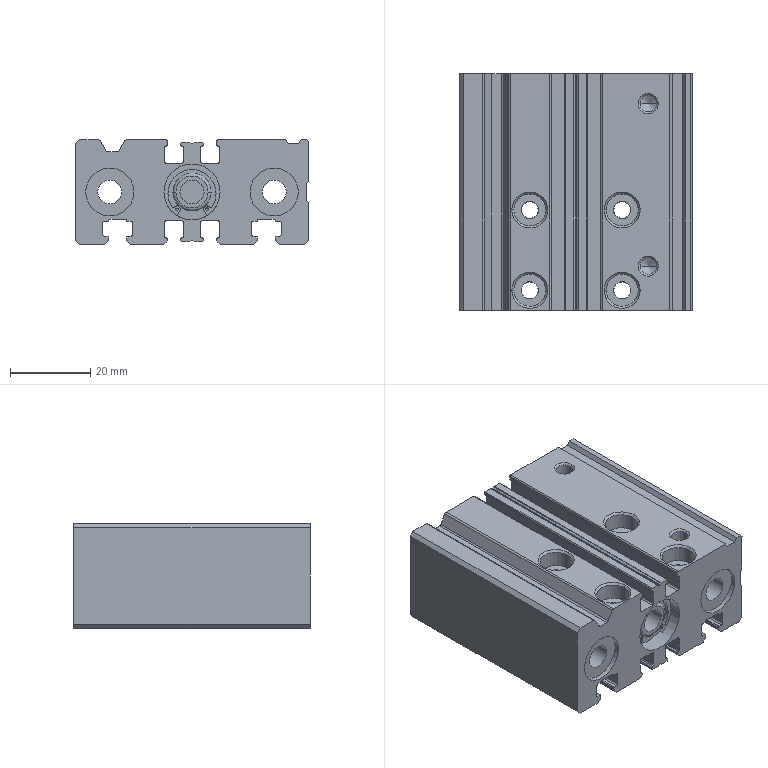Component | SolidWorks | TC_L_12x30_S_0-1_TC_L_12x3030_b-1 | 1 solid | 367 faces | box 58 x 59 x 26 mm | volume 60590 mm3 | cylinder 166 | plane 141 | cone 58 | torus 2 | commonest cylinder face diameters 0.8 x20 1 x18 0.4 x18 4.134 x16 3 x14 12 x12 0.6 x10 3.242 x8